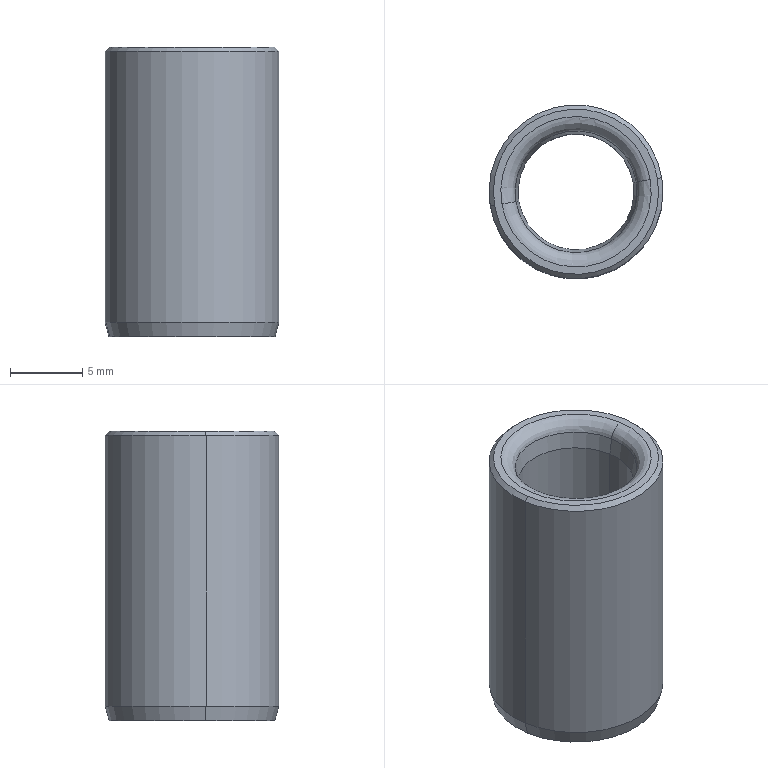Component | SolidWorks | MPBZ8_20-2 | 1 solid | 18 faces | box 12 x 12 x 20 mm | volume 1224 mm3 | cone 8 | cylinder 4 | torus 4 | plane 2 | commonest cylinder face diameters 12 x2 8 x2
build123d program:
from build123d import *


with BuildPart() as part:
    # Sketch1 → Revolve1 (revolve)
    with BuildSketch(Plane.XY, mode=Mode.PRIVATE) as revolve1_sk:
        with BuildLine():
            Line((0, 5.7), (0, 5.192))
            ThreePointArc((0, 5.192), (0.234, 4.549), (0.8264, 4.207))
            Line((0.8264, 4.207), (2, 4))
            Line((2, 4), (18, 4))
            Line((18, 4), (19.174, 4.207))
            ThreePointArc((19.174, 4.207), (19.766, 4.549), (20, 5.192))
            Line((20, 5.192), (20, 5.732))
            Line((20, 5.732), (19, 6))
            Line((19, 6), (0.3, 6))
            Line((0.3, 6), (0, 5.7))
        make_face()
    revolve(revolve1_sk.sketch.rotate(Axis((20, 0, 0), (-1, 0, 0)), 270), axis=Axis((20, 0, 0), (-1, 0, 0)))


solid = part.part

# Placed as in the assembly
solid = solid.moved(Location((-45.939, -84.245, 300), (0, 90, 0)))
STEP:
#1=CARTESIAN_POINT('',(-1.575,-3.279,11.063));
#2=VERTEX_POINT('',#1);
#3=CARTESIAN_POINT('',(-2.042,-3.355,11.063));
#4=VERTEX_POINT('',#3);
#5=CARTESIAN_POINT('',(-1.809,-3.317,11.063));
#6=DIRECTION('',(0.,0.,1.));
#7=DIRECTION('',(0.9869,0.1613,0.));
#8=AXIS2_PLACEMENT_3D('',#5,#6,#7);
#9=CIRCLE('',#8,0.2362);
#10=EDGE_CURVE('',#2,#4,#9,.T.);
#11=ORIENTED_EDGE('',*,*,#10,.T.);
#12=CARTESIAN_POINT('',(-2.042,-3.355,11.799));
#13=VERTEX_POINT('',#12);
#14=CARTESIAN_POINT('',(-2.042,-3.355,11.024));
#15=DIRECTION('',(0.,0.,1.));
#16=VECTOR('',#15,39.37);
#17=LINE('',#14,#16);
#18=EDGE_CURVE('',#4,#13,#17,.T.);
#19=ORIENTED_EDGE('',*,*,#18,.T.);
#20=CARTESIAN_POINT('',(-1.575,-3.279,11.799));
#21=VERTEX_POINT('',#20);
#22=CARTESIAN_POINT('',(-1.809,-3.317,11.799));
#23=DIRECTION('',(0.,0.,1.));
#24=DIRECTION('',(0.9869,0.1613,0.));
#25=AXIS2_PLACEMENT_3D('',#22,#23,#24);
#26=CIRCLE('',#25,0.2362);
#27=EDGE_CURVE('',#21,#13,#26,.T.);
#28=ORIENTED_EDGE('',*,*,#27,.F.);
#29=CARTESIAN_POINT('',(-1.575,-3.279,11.024));
#30=DIRECTION('',(0.,0.,1.));
#31=VECTOR('',#30,39.37);
#32=LINE('',#29,#31);
#33=EDGE_CURVE('',#2,#21,#32,.T.);
#34=ORIENTED_EDGE('',*,*,#33,.F.);
#35=EDGE_LOOP('',(#11,#19,#28,#34));
#36=FACE_OUTER_BOUND('',#35,.T.);
#37=CARTESIAN_POINT('',(-1.809,-3.317,11.024));
#38=DIRECTION('',(0.,0.,1.));
#39=DIRECTION('',(0.9869,0.1613,0.));
#40=AXIS2_PLACEMENT_3D('',#37,#38,#39);
#41=CYLINDRICAL_SURFACE('',#40,0.2362);
#42=ADVANCED_FACE('',(#36),#41,.T.);
#43=CARTESIAN_POINT('',(-1.586,-3.28,11.024));
#44=VERTEX_POINT('',#43);
#45=CARTESIAN_POINT('',(-2.031,-3.353,11.024));
#46=VERTEX_POINT('',#45);
#47=CARTESIAN_POINT('',(-1.809,-3.317,11.024));
#48=DIRECTION('',(0.,0.,1.));
#49=DIRECTION('',(0.9869,0.1613,0.));
#50=AXIS2_PLACEMENT_3D('',#47,#48,#49);
#51=CIRCLE('',#50,0.2257);
#52=EDGE_CURVE('',#44,#46,#51,.T.);
#53=ORIENTED_EDGE('',*,*,#52,.T.);
#54=CARTESIAN_POINT('',(-2.031,-3.353,11.024));
#55=DIRECTION('',(-0.2554,-0.04174,0.9659));
#56=VECTOR('',#55,39.37);
#57=LINE('',#54,#56);
#58=EDGE_CURVE('',#46,#4,#57,.T.);
#59=ORIENTED_EDGE('',*,*,#58,.T.);
#60=ORIENTED_EDGE('',*,*,#10,.F.);
#61=CARTESIAN_POINT('',(-1.586,-3.28,11.024));
#62=DIRECTION('',(0.2554,0.04174,0.9659));
#63=VECTOR('',#62,39.37);
#64=LINE('',#61,#63);
#65=EDGE_CURVE('',#44,#2,#64,.T.);
#66=ORIENTED_EDGE('',*,*,#65,.F.);
#67=EDGE_LOOP('',(#53,#59,#60,#66));
#68=FACE_OUTER_BOUND('',#67,.T.);
#69=CARTESIAN_POINT('',(-1.809,-3.317,11.024));
#70=DIRECTION('',(0.,0.,1.));
#71=DIRECTION('',(0.9869,0.1613,0.));
#72=AXIS2_PLACEMENT_3D('',#69,#70,#71);
#73=CONICAL_SURFACE('',#72,0.2257,0.2618);
#74=ADVANCED_FACE('',(#68),#73,.T.);
#75=CARTESIAN_POINT('',(-1.645,-3.29,11.056));
#76=VERTEX_POINT('',#75);
#77=CARTESIAN_POINT('',(-1.972,-3.343,11.056));
#78=VERTEX_POINT('',#77);
#79=CARTESIAN_POINT('',(-1.809,-3.317,11.056));
#80=DIRECTION('',(0.,0.,1.));
#81=DIRECTION('',(0.9869,0.1613,0.));
#82=AXIS2_PLACEMENT_3D('',#79,#80,#81);
#83=CIRCLE('',#82,0.1656);
#84=EDGE_CURVE('',#76,#78,#83,.T.);
#85=ORIENTED_EDGE('',*,*,#84,.T.);
#86=CARTESIAN_POINT('',(-2.01,-3.35,11.024));
#87=VERTEX_POINT('',#86);
#88=CARTESIAN_POINT('',(-2.01,-3.35,11.063));
#89=DIRECTION('',(-0.1613,0.9869,0.));
#90=DIRECTION('',(-0.9869,-0.1613,0.));
#91=AXIS2_PLACEMENT_3D('',#88,#89,#90);
#92=CIRCLE('',#91,0.03937);
#93=EDGE_CURVE('',#78,#87,#92,.T.);
#94=ORIENTED_EDGE('',*,*,#93,.T.);
#95=CARTESIAN_POINT('',(-1.607,-3.284,11.024));
#96=VERTEX_POINT('',#95);
#97=CARTESIAN_POINT('',(-1.809,-3.317,11.024));
#98=DIRECTION('',(0.,0.,1.));
#99=DIRECTION('',(0.9869,0.1613,0.));
#100=AXIS2_PLACEMENT_3D('',#97,#98,#99);
#101=CIRCLE('',#100,0.2044);
#102=EDGE_CURVE('',#96,#87,#101,.T.);
#103=ORIENTED_EDGE('',*,*,#102,.F.);
#104=CARTESIAN_POINT('',(-1.607,-3.284,11.063));
#105=DIRECTION('',(0.1613,-0.9869,0.));
#106=DIRECTION('',(0.9869,0.1613,0.));
#107=AXIS2_PLACEMENT_3D('',#104,#105,#106);
#108=CIRCLE('',#107,0.03937);
#109=EDGE_CURVE('',#76,#96,#108,.T.);
#110=ORIENTED_EDGE('',*,*,#109,.F.);
#111=EDGE_LOOP('',(#85,#94,#103,#110));
#112=FACE_OUTER_BOUND('',#111,.T.);
#113=CARTESIAN_POINT('',(-1.809,-3.317,11.063));
#114=DIRECTION('',(0.,0.,1.));
#115=DIRECTION('',(0.9869,0.1613,0.));
#116=AXIS2_PLACEMENT_3D('',#113,#114,#115);
#117=TOROIDAL_SURFACE('',#116,0.2044,0.03937);
#118=ADVANCED_FACE('',(#112),#117,.T.);
#119=CARTESIAN_POINT('',(-1.964,-3.342,11.102));
#120=VERTEX_POINT('',#119);
#121=CARTESIAN_POINT('',(-1.653,-3.291,11.102));
#122=VERTEX_POINT('',#121);
#123=CARTESIAN_POINT('',(-1.809,-3.317,11.102));
#124=DIRECTION('',(0.,0.,1.));
#125=DIRECTION('',(0.9869,0.1613,0.));
#126=AXIS2_PLACEMENT_3D('',#123,#124,#125);
#127=CIRCLE('',#126,0.1575);
#128=EDGE_CURVE('',#120,#122,#127,.T.);
#129=ORIENTED_EDGE('',*,*,#128,.T.);
#130=CARTESIAN_POINT('',(-1.653,-3.291,11.102));
#131=DIRECTION('',(0.1714,0.028,-0.9848));
#132=VECTOR('',#131,39.37);
#133=LINE('',#130,#132);
#134=EDGE_CURVE('',#122,#76,#133,.T.);
#135=ORIENTED_EDGE('',*,*,#134,.T.);
#136=CARTESIAN_POINT('',(-1.809,-3.317,11.056));
#137=DIRECTION('',(0.,0.,1.));
#138=DIRECTION('',(0.9869,0.1613,0.));
#139=AXIS2_PLACEMENT_3D('',#136,#137,#138);
#140=CIRCLE('',#139,0.1656);
#141=EDGE_CURVE('',#78,#76,#140,.T.);
#142=ORIENTED_EDGE('',*,*,#141,.F.);
#143=CARTESIAN_POINT('',(-1.964,-3.342,11.102));
#144=DIRECTION('',(-0.1714,-0.028,-0.9848));
#145=VECTOR('',#144,39.37);
#146=LINE('',#143,#145);
#147=EDGE_CURVE('',#120,#78,#146,.T.);
#148=ORIENTED_EDGE('',*,*,#147,.F.);
#149=EDGE_LOOP('',(#129,#135,#142,#148));
#150=FACE_OUTER_BOUND('',#149,.T.);
#151=CARTESIAN_POINT('',(-1.809,-3.317,11.102));
#152=DIRECTION('',(0.,0.,-1.));
#153=DIRECTION('',(-0.9869,-0.1613,0.));
#154=AXIS2_PLACEMENT_3D('',#151,#152,#153);
#155=CONICAL_SURFACE('',#154,0.1575,0.1745);
#156=ADVANCED_FACE('',(#150),#155,.F.);
#157=ORIENTED_EDGE('',*,*,#128,.F.);
#158=CARTESIAN_POINT('',(-1.964,-3.342,11.732));
#159=VERTEX_POINT('',#158);
#160=CARTESIAN_POINT('',(-1.964,-3.342,11.024));
#161=DIRECTION('',(0.,0.,1.));
#162=VECTOR('',#161,39.37);
#163=LINE('',#160,#162);
#164=EDGE_CURVE('',#120,#159,#163,.T.);
#165=ORIENTED_EDGE('',*,*,#164,.T.);
#166=CARTESIAN_POINT('',(-1.653,-3.291,11.732));
#167=VERTEX_POINT('',#166);
#168=CARTESIAN_POINT('',(-1.809,-3.317,11.732));
#169=DIRECTION('',(0.,0.,1.));
#170=DIRECTION('',(0.9869,0.1613,0.));
#171=AXIS2_PLACEMENT_3D('',#168,#169,#170);
#172=CIRCLE('',#171,0.1575);
#173=EDGE_CURVE('',#159,#167,#172,.T.);
#174=ORIENTED_EDGE('',*,*,#173,.T.);
#175=CARTESIAN_POINT('',(-1.653,-3.291,11.024));
#176=DIRECTION('',(0.,0.,1.));
#177=VECTOR('',#176,39.37);
#178=LINE('',#175,#177);
#179=EDGE_CURVE('',#122,#167,#178,.T.);
#180=ORIENTED_EDGE('',*,*,#179,.F.);
#181=EDGE_LOOP('',(#157,#165,#174,#180));
#182=FACE_OUTER_BOUND('',#181,.T.);
#183=CARTESIAN_POINT('',(-1.809,-3.317,11.024));
#184=DIRECTION('',(0.,0.,1.));
#185=DIRECTION('',(0.9869,0.1613,0.));
#186=AXIS2_PLACEMENT_3D('',#183,#184,#185);
#187=CYLINDRICAL_SURFACE('',#186,0.1575);
#188=ADVANCED_FACE('',(#182),#187,.F.);
#189=ORIENTED_EDGE('',*,*,#173,.F.);
#190=CARTESIAN_POINT('',(-1.972,-3.343,11.778));
#191=VERTEX_POINT('',#190);
#192=CARTESIAN_POINT('',(-1.972,-3.343,11.778));
#193=DIRECTION('',(-0.1714,-0.028,0.9848));
#194=VECTOR('',#193,39.37);
#195=LINE('',#192,#194);
#196=EDGE_CURVE('',#159,#191,#195,.T.);
#197=ORIENTED_EDGE('',*,*,#196,.T.);
#198=CARTESIAN_POINT('',(-1.645,-3.29,11.778));
#199=VERTEX_POINT('',#198);
#200=CARTESIAN_POINT('',(-1.809,-3.317,11.778));
#201=DIRECTION('',(0.,0.,1.));
#202=DIRECTION('',(0.9869,0.1613,0.));
#203=AXIS2_PLACEMENT_3D('',#200,#201,#202);
#204=CIRCLE('',#203,0.1656);
#205=EDGE_CURVE('',#191,#199,#204,.T.);
#206=ORIENTED_EDGE('',*,*,#205,.T.);
#207=CARTESIAN_POINT('',(-1.645,-3.29,11.778));
#208=DIRECTION('',(0.1714,0.028,0.9848));
#209=VECTOR('',#208,39.37);
#210=LINE('',#207,#209);
#211=EDGE_CURVE('',#167,#199,#210,.T.);
#212=ORIENTED_EDGE('',*,*,#211,.F.);
#213=EDGE_LOOP('',(#189,#197,#206,#212));
#214=FACE_OUTER_BOUND('',#213,.T.);
#215=CARTESIAN_POINT('',(-1.809,-3.317,11.778));
#216=DIRECTION('',(0.,0.,1.));
#217=DIRECTION('',(0.9869,0.1613,0.));
#218=AXIS2_PLACEMENT_3D('',#215,#216,#217);
#219=CONICAL_SURFACE('',#218,0.1656,0.1745);
#220=ADVANCED_FACE('',(#214),#219,.F.);
#221=CARTESIAN_POINT('',(-1.607,-3.284,11.811));
#222=VERTEX_POINT('',#221);
#223=CARTESIAN_POINT('',(-2.01,-3.35,11.811));
#224=VERTEX_POINT('',#223);
#225=CARTESIAN_POINT('',(-1.809,-3.317,11.811));
#226=DIRECTION('',(0.,0.,1.));
#227=DIRECTION('',(0.9869,0.1613,0.));
#228=AXIS2_PLACEMENT_3D('',#225,#226,#227);
#229=CIRCLE('',#228,0.2044);
#230=EDGE_CURVE('',#222,#224,#229,.T.);
#231=ORIENTED_EDGE('',*,*,#230,.T.);
#232=CARTESIAN_POINT('',(-2.01,-3.35,11.772));
#233=DIRECTION('',(-0.1613,0.9869,0.));
#234=DIRECTION('',(-0.9869,-0.1613,0.));
#235=AXIS2_PLACEMENT_3D('',#232,#233,#234);
#236=CIRCLE('',#235,0.03937);
#237=EDGE_CURVE('',#224,#191,#236,.T.);
#238=ORIENTED_EDGE('',*,*,#237,.T.);
#239=CARTESIAN_POINT('',(-1.809,-3.317,11.778));
#240=DIRECTION('',(0.,0.,1.));
#241=DIRECTION('',(0.9869,0.1613,0.));
#242=AXIS2_PLACEMENT_3D('',#239,#240,#241);
#243=CIRCLE('',#242,0.1656);
#244=EDGE_CURVE('',#199,#191,#243,.T.);
#245=ORIENTED_EDGE('',*,*,#244,.F.);
#246=CARTESIAN_POINT('',(-1.607,-3.284,11.772));
#247=DIRECTION('',(0.1613,-0.9869,0.));
#248=DIRECTION('',(0.9869,0.1613,0.));
#249=AXIS2_PLACEMENT_3D('',#246,#247,#248);
#250=CIRCLE('',#249,0.03937);
#251=EDGE_CURVE('',#222,#199,#250,.T.);
#252=ORIENTED_EDGE('',*,*,#251,.F.);
#253=EDGE_LOOP('',(#231,#238,#245,#252));
#254=FACE_OUTER_BOUND('',#253,.T.);
#255=CARTESIAN_POINT('',(-1.809,-3.317,11.772));
#256=DIRECTION('',(0.,0.,1.));
#257=DIRECTION('',(0.9869,0.1613,0.));
#258=AXIS2_PLACEMENT_3D('',#255,#256,#257);
#259=TOROIDAL_SURFACE('',#258,0.2044,0.03937);
#260=ADVANCED_FACE('',(#254),#259,.T.);
#261=CARTESIAN_POINT('',(-1.587,-3.281,11.811));
#262=VERTEX_POINT('',#261);
#263=CARTESIAN_POINT('',(-2.03,-3.353,11.811));
#264=VERTEX_POINT('',#263);
#265=CARTESIAN_POINT('',(-1.809,-3.317,11.811));
#266=DIRECTION('',(0.,0.,1.));
#267=DIRECTION('',(0.9869,0.1613,0.));
#268=AXIS2_PLACEMENT_3D('',#265,#266,#267);
#269=CIRCLE('',#268,0.2244);
#270=EDGE_CURVE('',#262,#264,#269,.T.);
#271=ORIENTED_EDGE('',*,*,#270,.F.);
#272=CARTESIAN_POINT('',(-1.575,-3.279,11.799));
#273=DIRECTION('',(0.6979,0.114,-0.7071));
#274=VECTOR('',#273,39.37);
#275=LINE('',#272,#274);
#276=EDGE_CURVE('',#262,#21,#275,.T.);
#277=ORIENTED_EDGE('',*,*,#276,.T.);
#278=ORIENTED_EDGE('',*,*,#27,.T.);
#279=CARTESIAN_POINT('',(-2.042,-3.355,11.799));
#280=DIRECTION('',(-0.6979,-0.114,-0.7071));
#281=VECTOR('',#280,39.37);
#282=LINE('',#279,#281);
#283=EDGE_CURVE('',#264,#13,#282,.T.);
#284=ORIENTED_EDGE('',*,*,#283,.F.);
#285=EDGE_LOOP('',(#271,#277,#278,#284));
#286=FACE_OUTER_BOUND('',#285,.T.);
#287=CARTESIAN_POINT('',(-1.809,-3.317,11.799));
#288=DIRECTION('',(0.,0.,-1.));
#289=DIRECTION('',(-0.9869,-0.1613,0.));
#290=AXIS2_PLACEMENT_3D('',#287,#288,#289);
#291=CONICAL_SURFACE('',#290,0.2362,0.7854);
#292=ADVANCED_FACE('',(#286),#291,.T.);
#293=ORIENTED_EDGE('',*,*,#276,.F.);
#294=CARTESIAN_POINT('',(-1.809,-3.317,11.811));
#295=DIRECTION('',(0.,0.,1.));
#296=DIRECTION('',(0.9869,0.1613,0.));
#297=AXIS2_PLACEMENT_3D('',#294,#295,#296);
#298=CIRCLE('',#297,0.2244);
#299=EDGE_CURVE('',#264,#262,#298,.T.);
#300=ORIENTED_EDGE('',*,*,#299,.F.);
#301=ORIENTED_EDGE('',*,*,#283,.T.);
#302=CARTESIAN_POINT('',(-1.809,-3.317,11.799));
#303=DIRECTION('',(0.,0.,1.));
#304=DIRECTION('',(0.9869,0.1613,0.));
#305=AXIS2_PLACEMENT_3D('',#302,#303,#304);
#306=CIRCLE('',#305,0.2362);
#307=EDGE_CURVE('',#13,#21,#306,.T.);
#308=ORIENTED_EDGE('',*,*,#307,.T.);
#309=EDGE_LOOP('',(#293,#300,#301,#308));
#310=FACE_OUTER_BOUND('',#309,.T.);
#311=CARTESIAN_POINT('',(-1.809,-3.317,11.799));
#312=DIRECTION('',(0.,0.,-1.));
#313=DIRECTION('',(-0.9869,-0.1613,0.));
#314=AXIS2_PLACEMENT_3D('',#311,#312,#313);
#315=CONICAL_SURFACE('',#314,0.2362,0.7854);
#316=ADVANCED_FACE('',(#310),#315,.T.);
#317=ORIENTED_EDGE('',*,*,#230,.F.);
#318=CARTESIAN_POINT('',(-1.809,-3.317,11.811));
#319=DIRECTION('',(0.,0.,1.));
#320=DIRECTION('',(0.9869,0.1613,0.));
#321=AXIS2_PLACEMENT_3D('',#318,#319,#320);
#322=CIRCLE('',#321,0.2044);
#323=EDGE_CURVE('',#224,#222,#322,.T.);
#324=ORIENTED_EDGE('',*,*,#323,.F.);
#325=EDGE_LOOP('',(#317,#324));
#326=FACE_BOUND('',#325,.T.);
#327=ORIENTED_EDGE('',*,*,#299,.T.);
#328=ORIENTED_EDGE('',*,*,#270,.T.);
#329=EDGE_LOOP('',(#327,#328));
#330=FACE_OUTER_BOUND('',#329,.T.);
#331=CARTESIAN_POINT('',(-1.845,-3.095,11.811));
#332=DIRECTION('',(0.,0.,-1.));
#333=DIRECTION('',(-0.9869,-0.1613,0.));
#334=AXIS2_PLACEMENT_3D('',#331,#332,#333);
#335=PLANE('',#334);
#336=ADVANCED_FACE('',(#326,#330),#335,.F.);
#337=ORIENTED_EDGE('',*,*,#237,.F.);
#338=ORIENTED_EDGE('',*,*,#323,.T.);
#339=ORIENTED_EDGE('',*,*,#251,.T.);
#340=ORIENTED_EDGE('',*,*,#205,.F.);
#341=EDGE_LOOP('',(#337,#338,#339,#340));
#342=FACE_OUTER_BOUND('',#341,.T.);
#343=CARTESIAN_POINT('',(-1.809,-3.317,11.772));
#344=DIRECTION('',(0.,0.,1.));
#345=DIRECTION('',(0.9869,0.1613,0.));
#346=AXIS2_PLACEMENT_3D('',#343,#344,#345);
#347=TOROIDAL_SURFACE('',#346,0.2044,0.03937);
#348=ADVANCED_FACE('',(#342),#347,.T.);
#349=ORIENTED_EDGE('',*,*,#196,.F.);
#350=CARTESIAN_POINT('',(-1.809,-3.317,11.732));
#351=DIRECTION('',(0.,0.,1.));
#352=DIRECTION('',(0.9869,0.1613,0.));
#353=AXIS2_PLACEMENT_3D('',#350,#351,#352);
#354=CIRCLE('',#353,0.1575);
#355=EDGE_CURVE('',#167,#159,#354,.T.);
#356=ORIENTED_EDGE('',*,*,#355,.F.);
#357=ORIENTED_EDGE('',*,*,#211,.T.);
#358=ORIENTED_EDGE('',*,*,#244,.T.);
#359=EDGE_LOOP('',(#349,#356,#357,#358));
#360=FACE_OUTER_BOUND('',#359,.T.);
#361=CARTESIAN_POINT('',(-1.809,-3.317,11.778));
#362=DIRECTION('',(0.,0.,1.));
#363=DIRECTION('',(0.9869,0.1613,0.));
#364=AXIS2_PLACEMENT_3D('',#361,#362,#363);
#365=CONICAL_SURFACE('',#364,0.1656,0.1745);
#366=ADVANCED_FACE('',(#360),#365,.F.);
#367=ORIENTED_EDGE('',*,*,#164,.F.);
#368=CARTESIAN_POINT('',(-1.809,-3.317,11.102));
#369=DIRECTION('',(0.,0.,1.));
#370=DIRECTION('',(0.9869,0.1613,0.));
#371=AXIS2_PLACEMENT_3D('',#368,#369,#370);
#372=CIRCLE('',#371,0.1575);
#373=EDGE_CURVE('',#122,#120,#372,.T.);
#374=ORIENTED_EDGE('',*,*,#373,.F.);
#375=ORIENTED_EDGE('',*,*,#179,.T.);
#376=ORIENTED_EDGE('',*,*,#355,.T.);
#377=EDGE_LOOP('',(#367,#374,#375,#376));
#378=FACE_OUTER_BOUND('',#377,.T.);
#379=CARTESIAN_POINT('',(-1.809,-3.317,11.024));
#380=DIRECTION('',(0.,0.,1.));
#381=DIRECTION('',(0.9869,0.1613,0.));
#382=AXIS2_PLACEMENT_3D('',#379,#380,#381);
#383=CYLINDRICAL_SURFACE('',#382,0.1575);
#384=ADVANCED_FACE('',(#378),#383,.F.);
#385=ORIENTED_EDGE('',*,*,#134,.F.);
#386=ORIENTED_EDGE('',*,*,#373,.T.);
#387=ORIENTED_EDGE('',*,*,#147,.T.);
#388=ORIENTED_EDGE('',*,*,#84,.F.);
#389=EDGE_LOOP('',(#385,#386,#387,#388));
#390=FACE_OUTER_BOUND('',#389,.T.);
#391=CARTESIAN_POINT('',(-1.809,-3.317,11.102));
#392=DIRECTION('',(0.,0.,-1.));
#393=DIRECTION('',(-0.9869,-0.1613,0.));
#394=AXIS2_PLACEMENT_3D('',#391,#392,#393);
#395=CONICAL_SURFACE('',#394,0.1575,0.1745);
#396=ADVANCED_FACE('',(#390),#395,.F.);
#397=ORIENTED_EDGE('',*,*,#93,.F.);
#398=ORIENTED_EDGE('',*,*,#141,.T.);
#399=ORIENTED_EDGE('',*,*,#109,.T.);
#400=CARTESIAN_POINT('',(-1.809,-3.317,11.024));
#401=DIRECTION('',(0.,0.,1.));
#402=DIRECTION('',(0.9869,0.1613,0.));
#403=AXIS2_PLACEMENT_3D('',#400,#401,#402);
#404=CIRCLE('',#403,0.2044);
#405=EDGE_CURVE('',#87,#96,#404,.T.);
#406=ORIENTED_EDGE('',*,*,#405,.F.);
#407=EDGE_LOOP('',(#397,#398,#399,#406));
#408=FACE_OUTER_BOUND('',#407,.T.);
#409=CARTESIAN_POINT('',(-1.809,-3.317,11.063));
#410=DIRECTION('',(0.,0.,1.));
#411=DIRECTION('',(0.9869,0.1613,0.));
#412=AXIS2_PLACEMENT_3D('',#409,#410,#411);
#413=TOROIDAL_SURFACE('',#412,0.2044,0.03937);
#414=ADVANCED_FACE('',(#408),#413,.T.);
#415=ORIENTED_EDGE('',*,*,#52,.F.);
#416=CARTESIAN_POINT('',(-1.809,-3.317,11.024));
#417=DIRECTION('',(0.,0.,1.));
#418=DIRECTION('',(0.9869,0.1613,0.));
#419=AXIS2_PLACEMENT_3D('',#416,#417,#418);
#420=CIRCLE('',#419,0.2257);
#421=EDGE_CURVE('',#46,#44,#420,.T.);
#422=ORIENTED_EDGE('',*,*,#421,.F.);
#423=EDGE_LOOP('',(#415,#422));
#424=FACE_OUTER_BOUND('',#423,.T.);
#425=ORIENTED_EDGE('',*,*,#102,.T.);
#426=ORIENTED_EDGE('',*,*,#405,.T.);
#427=EDGE_LOOP('',(#425,#426));
#428=FACE_BOUND('',#427,.T.);
#429=CARTESIAN_POINT('',(-1.842,-3.115,11.024));
#430=DIRECTION('',(0.,0.,1.));
#431=DIRECTION('',(0.9869,0.1613,0.));
#432=AXIS2_PLACEMENT_3D('',#429,#430,#431);
#433=PLANE('',#432);
#434=ADVANCED_FACE('',(#424,#428),#433,.F.);
#435=ORIENTED_EDGE('',*,*,#58,.F.);
#436=ORIENTED_EDGE('',*,*,#421,.T.);
#437=ORIENTED_EDGE('',*,*,#65,.T.);
#438=CARTESIAN_POINT('',(-1.809,-3.317,11.063));
#439=DIRECTION('',(0.,0.,1.));
#440=DIRECTION('',(0.9869,0.1613,0.));
#441=AXIS2_PLACEMENT_3D('',#438,#439,#440);
#442=CIRCLE('',#441,0.2362);
#443=EDGE_CURVE('',#4,#2,#442,.T.);
#444=ORIENTED_EDGE('',*,*,#443,.F.);
#445=EDGE_LOOP('',(#435,#436,#437,#444));
#446=FACE_OUTER_BOUND('',#445,.T.);
#447=CARTESIAN_POINT('',(-1.809,-3.317,11.024));
#448=DIRECTION('',(0.,0.,1.));
#449=DIRECTION('',(0.9869,0.1613,0.));
#450=AXIS2_PLACEMENT_3D('',#447,#448,#449);
#451=CONICAL_SURFACE('',#450,0.2257,0.2618);
#452=ADVANCED_FACE('',(#446),#451,.T.);
#453=ORIENTED_EDGE('',*,*,#18,.F.);
#454=ORIENTED_EDGE('',*,*,#443,.T.);
#455=ORIENTED_EDGE('',*,*,#33,.T.);
#456=ORIENTED_EDGE('',*,*,#307,.F.);
#457=EDGE_LOOP('',(#453,#454,#455,#456));
#458=FACE_OUTER_BOUND('',#457,.T.);
#459=CARTESIAN_POINT('',(-1.809,-3.317,11.024));
#460=DIRECTION('',(0.,0.,1.));
#461=DIRECTION('',(0.9869,0.1613,0.));
#462=AXIS2_PLACEMENT_3D('',#459,#460,#461);
#463=CYLINDRICAL_SURFACE('',#462,0.2362);
#464=ADVANCED_FACE('',(#458),#463,.T.);
#465=CLOSED_SHELL('',(#42,#74,#118,#156,#188,#220,#260,#292,#316,#336,#348,#366,#384,#396,#414,#434,#452,#464));
#466=MANIFOLD_SOLID_BREP('',#465);
#467=CARTESIAN_POINT('',(0.,0.,0.));
#468=DIRECTION('',(0.,0.,1.));
#469=DIRECTION('',(1.,0.,0.));
#470=AXIS2_PLACEMENT_3D('',#467,#468,#469);
#471=(LENGTH_UNIT()NAMED_UNIT(*)SI_UNIT($,.METRE.));
#472=LENGTH_MEASURE_WITH_UNIT(LENGTH_MEASURE(0.0254),#471);
#473=DIMENSIONAL_EXPONENTS(1.,0.,0.,0.,0.,0.,0.);
#474=(CONVERSION_BASED_UNIT('',#472)LENGTH_UNIT()NAMED_UNIT(#473));
#475=UNCERTAINTY_MEASURE_WITH_UNIT(LENGTH_MEASURE(0.00001),#474,'','');
#476=(NAMED_UNIT(*)PLANE_ANGLE_UNIT()SI_UNIT($,.RADIAN.));
#477=(NAMED_UNIT(*)SI_UNIT($,.STERADIAN.)SOLID_ANGLE_UNIT());
#478=(GEOMETRIC_REPRESENTATION_CONTEXT(3)GLOBAL_UNCERTAINTY_ASSIGNED_CONTEXT((#475))GLOBAL_UNIT_ASSIGNED_CONTEXT((#474,#476,#477))REPRESENTATION_CONTEXT('',''));
#479=ADVANCED_BREP_SHAPE_REPRESENTATION('',(#466,#470),#478);
#480=COLOUR_RGB('',0.7922,0.8196,0.9333);
#481=FILL_AREA_STYLE_COLOUR('',#480);
#482=FILL_AREA_STYLE('',(#481));
#483=SURFACE_STYLE_FILL_AREA(#482);
#484=SURFACE_SIDE_STYLE('',(#483));
#485=SURFACE_STYLE_USAGE(.BOTH.,#484);
#486=PRESENTATION_STYLE_ASSIGNMENT((#485));
#487=STYLED_ITEM('',(#486),#466);
#488=PRESENTATION_LAYER_ASSIGNMENT('','',(#487));
#489=(LENGTH_UNIT()NAMED_UNIT(*)SI_UNIT($,.METRE.));
#490=LENGTH_MEASURE_WITH_UNIT(LENGTH_MEASURE(0.0254),#489);
#491=DIMENSIONAL_EXPONENTS(1.,0.,0.,0.,0.,0.,0.);
#492=(CONVERSION_BASED_UNIT('',#490)LENGTH_UNIT()NAMED_UNIT(#491));
#493=UNCERTAINTY_MEASURE_WITH_UNIT(LENGTH_MEASURE(0.00001),#492,'','');
#494=(NAMED_UNIT(*)PLANE_ANGLE_UNIT()SI_UNIT($,.RADIAN.));
#495=(NAMED_UNIT(*)SI_UNIT($,.STERADIAN.)SOLID_ANGLE_UNIT());
#496=(GEOMETRIC_REPRESENTATION_CONTEXT(3)GLOBAL_UNCERTAINTY_ASSIGNED_CONTEXT((#493))GLOBAL_UNIT_ASSIGNED_CONTEXT((#492,#494,#495))REPRESENTATION_CONTEXT('',''));
#497=MECHANICAL_DESIGN_GEOMETRIC_PRESENTATION_REPRESENTATION('',(#487),#496);